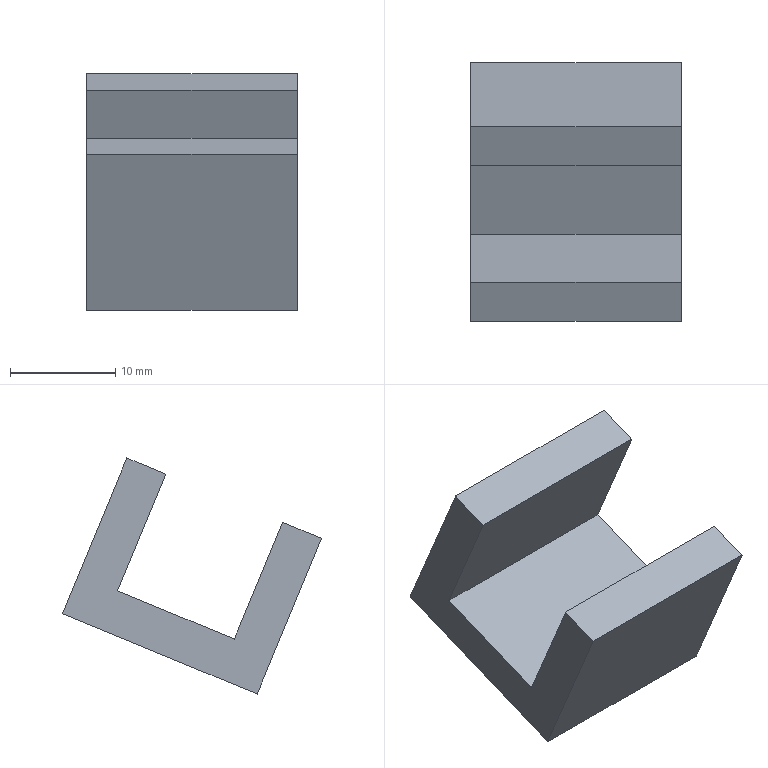Component | SolidWorks | 2026.08.03FixedRail-1 | 1 solid | 10 faces | box 20 x 24.59 x 22.42 mm | volume 3520 mm3 | plane 10
build123d program:
from build123d import *

# Parameters (mm, degrees)
BOSS_EXTRUDE2_DEPTH = 10


with BuildPart() as part:
    # Sketch1 → Boss-Extrude2 (new, symmetric)
    with BuildSketch(Plane(origin=(0, 0, 0), x_dir=(0, 0, -1), z_dir=(1, 0, 0))):
        Polygon((-16, 10), (0, 10), (0, -10), (-16, -10), (-16, -6), (-4, -6), (-4, 6), (-16, 6), align=None)
    extrude(amount=BOSS_EXTRUDE2_DEPTH, both=True)


solid = part.part

# Placed as in the assembly
solid = solid.moved(Location((80.094, 7.464, 7.823), (22.448, 0, 0)))
STEP:
#1=COLOUR_RGB('',0.7922,0.8196,0.9333);
#2=FILL_AREA_STYLE_COLOUR('',#1);
#3=FILL_AREA_STYLE('',(#2));
#4=SURFACE_STYLE_FILL_AREA(#3);
#5=SURFACE_SIDE_STYLE('',(#4));
#6=SURFACE_STYLE_USAGE(.BOTH.,#5);
#7=PRESENTATION_STYLE_ASSIGNMENT((#6));
#8=CARTESIAN_POINT('',(2.76,0.4172,1.041));
#9=VERTEX_POINT('',#8);
#10=CARTESIAN_POINT('',(2.76,0.2716,0.9804));
#11=VERTEX_POINT('',#10);
#12=CARTESIAN_POINT('',(2.76,0.4172,1.041));
#13=DIRECTION('',(0.,-0.9242,-0.3818));
#14=VECTOR('',#13,39.37);
#15=LINE('',#12,#14);
#16=EDGE_CURVE('',#9,#11,#15,.T.);
#17=ORIENTED_EDGE('',*,*,#16,.T.);
#18=CARTESIAN_POINT('',(3.547,0.2716,0.9804));
#19=VERTEX_POINT('',#18);
#20=CARTESIAN_POINT('',(3.547,0.2716,0.9804));
#21=DIRECTION('',(-1.,0.,0.));
#22=VECTOR('',#21,39.37);
#23=LINE('',#20,#22);
#24=EDGE_CURVE('',#19,#11,#23,.T.);
#25=ORIENTED_EDGE('',*,*,#24,.F.);
#26=CARTESIAN_POINT('',(3.547,0.4172,1.041));
#27=VERTEX_POINT('',#26);
#28=CARTESIAN_POINT('',(3.547,0.4172,1.041));
#29=DIRECTION('',(0.,-0.9242,-0.3818));
#30=VECTOR('',#29,39.37);
#31=LINE('',#28,#30);
#32=EDGE_CURVE('',#27,#19,#31,.T.);
#33=ORIENTED_EDGE('',*,*,#32,.F.);
#34=CARTESIAN_POINT('',(3.547,0.4172,1.041));
#35=DIRECTION('',(-1.,0.,0.));
#36=VECTOR('',#35,39.37);
#37=LINE('',#34,#36);
#38=EDGE_CURVE('',#27,#9,#37,.T.);
#39=ORIENTED_EDGE('',*,*,#38,.T.);
#40=EDGE_LOOP('',(#17,#25,#33,#39));
#41=FACE_OUTER_BOUND('',#40,.T.);
#42=CARTESIAN_POINT('',(3.547,0.4172,1.041));
#43=DIRECTION('',(0.,0.3818,-0.9242));
#44=DIRECTION('',(-1.,0.,0.));
#45=AXIS2_PLACEMENT_3D('',#42,#43,#44);
#46=PLANE('',#45);
#47=ADVANCED_FACE('',(#41),#46,.F.);
#48=CARTESIAN_POINT('',(2.76,0.452,0.5437));
#49=VERTEX_POINT('',#48);
#50=CARTESIAN_POINT('',(2.76,0.2716,0.9804));
#51=DIRECTION('',(0.,0.3818,-0.9242));
#52=VECTOR('',#51,39.37);
#53=LINE('',#50,#52);
#54=EDGE_CURVE('',#11,#49,#53,.T.);
#55=ORIENTED_EDGE('',*,*,#54,.T.);
#56=CARTESIAN_POINT('',(3.547,0.452,0.5437));
#57=VERTEX_POINT('',#56);
#58=CARTESIAN_POINT('',(3.547,0.452,0.5437));
#59=DIRECTION('',(-1.,0.,0.));
#60=VECTOR('',#59,39.37);
#61=LINE('',#58,#60);
#62=EDGE_CURVE('',#57,#49,#61,.T.);
#63=ORIENTED_EDGE('',*,*,#62,.F.);
#64=CARTESIAN_POINT('',(3.547,0.2716,0.9804));
#65=DIRECTION('',(0.,0.3818,-0.9242));
#66=VECTOR('',#65,39.37);
#67=LINE('',#64,#66);
#68=EDGE_CURVE('',#19,#57,#67,.T.);
#69=ORIENTED_EDGE('',*,*,#68,.F.);
#70=ORIENTED_EDGE('',*,*,#24,.T.);
#71=EDGE_LOOP('',(#55,#63,#69,#70));
#72=FACE_OUTER_BOUND('',#71,.T.);
#73=CARTESIAN_POINT('',(3.547,0.2716,0.9804));
#74=DIRECTION('',(0.,0.9242,0.3818));
#75=DIRECTION('',(0.,-0.3818,0.9242));
#76=AXIS2_PLACEMENT_3D('',#73,#74,#75);
#77=PLANE('',#76);
#78=ADVANCED_FACE('',(#72),#77,.F.);
#79=CARTESIAN_POINT('',(2.76,0.01541,0.3633));
#80=VERTEX_POINT('',#79);
#81=CARTESIAN_POINT('',(2.76,0.452,0.5437));
#82=DIRECTION('',(0.,-0.9242,-0.3818));
#83=VECTOR('',#82,39.37);
#84=LINE('',#81,#83);
#85=EDGE_CURVE('',#49,#80,#84,.T.);
#86=ORIENTED_EDGE('',*,*,#85,.T.);
#87=CARTESIAN_POINT('',(3.547,0.01541,0.3633));
#88=VERTEX_POINT('',#87);
#89=CARTESIAN_POINT('',(3.547,0.01541,0.3633));
#90=DIRECTION('',(-1.,0.,0.));
#91=VECTOR('',#90,39.37);
#92=LINE('',#89,#91);
#93=EDGE_CURVE('',#88,#80,#92,.T.);
#94=ORIENTED_EDGE('',*,*,#93,.F.);
#95=CARTESIAN_POINT('',(3.547,0.452,0.5437));
#96=DIRECTION('',(0.,-0.9242,-0.3818));
#97=VECTOR('',#96,39.37);
#98=LINE('',#95,#97);
#99=EDGE_CURVE('',#57,#88,#98,.T.);
#100=ORIENTED_EDGE('',*,*,#99,.F.);
#101=ORIENTED_EDGE('',*,*,#62,.T.);
#102=EDGE_LOOP('',(#86,#94,#100,#101));
#103=FACE_OUTER_BOUND('',#102,.T.);
#104=CARTESIAN_POINT('',(3.547,0.452,0.5437));
#105=DIRECTION('',(0.,0.3818,-0.9242));
#106=DIRECTION('',(0.,0.9242,0.3818));
#107=AXIS2_PLACEMENT_3D('',#104,#105,#106);
#108=PLANE('',#107);
#109=ADVANCED_FACE('',(#103),#108,.F.);
#110=CARTESIAN_POINT('',(2.76,-0.165,0.8));
#111=VERTEX_POINT('',#110);
#112=CARTESIAN_POINT('',(2.76,0.01541,0.3633));
#113=DIRECTION('',(0.,-0.3818,0.9242));
#114=VECTOR('',#113,39.37);
#115=LINE('',#112,#114);
#116=EDGE_CURVE('',#80,#111,#115,.T.);
#117=ORIENTED_EDGE('',*,*,#116,.T.);
#118=CARTESIAN_POINT('',(3.547,-0.165,0.8));
#119=VERTEX_POINT('',#118);
#120=CARTESIAN_POINT('',(3.547,-0.165,0.8));
#121=DIRECTION('',(-1.,0.,0.));
#122=VECTOR('',#121,39.37);
#123=LINE('',#120,#122);
#124=EDGE_CURVE('',#119,#111,#123,.T.);
#125=ORIENTED_EDGE('',*,*,#124,.F.);
#126=CARTESIAN_POINT('',(3.547,0.01541,0.3633));
#127=DIRECTION('',(0.,-0.3818,0.9242));
#128=VECTOR('',#127,39.37);
#129=LINE('',#126,#128);
#130=EDGE_CURVE('',#88,#119,#129,.T.);
#131=ORIENTED_EDGE('',*,*,#130,.F.);
#132=ORIENTED_EDGE('',*,*,#93,.T.);
#133=EDGE_LOOP('',(#117,#125,#131,#132));
#134=FACE_OUTER_BOUND('',#133,.T.);
#135=CARTESIAN_POINT('',(3.547,0.01541,0.3633));
#136=DIRECTION('',(0.,-0.9242,-0.3818));
#137=DIRECTION('',(0.,0.3818,-0.9242));
#138=AXIS2_PLACEMENT_3D('',#135,#136,#137);
#139=PLANE('',#138);
#140=ADVANCED_FACE('',(#134),#139,.F.);
#141=CARTESIAN_POINT('',(2.76,-0.3105,0.7399));
#142=VERTEX_POINT('',#141);
#143=CARTESIAN_POINT('',(2.76,-0.165,0.8));
#144=DIRECTION('',(0.,-0.9242,-0.3818));
#145=VECTOR('',#144,39.37);
#146=LINE('',#143,#145);
#147=EDGE_CURVE('',#111,#142,#146,.T.);
#148=ORIENTED_EDGE('',*,*,#147,.T.);
#149=CARTESIAN_POINT('',(3.547,-0.3105,0.7399));
#150=VERTEX_POINT('',#149);
#151=CARTESIAN_POINT('',(3.547,-0.3105,0.7399));
#152=DIRECTION('',(-1.,0.,0.));
#153=VECTOR('',#152,39.37);
#154=LINE('',#151,#153);
#155=EDGE_CURVE('',#150,#142,#154,.T.);
#156=ORIENTED_EDGE('',*,*,#155,.F.);
#157=CARTESIAN_POINT('',(3.547,-0.165,0.8));
#158=DIRECTION('',(0.,-0.9242,-0.3818));
#159=VECTOR('',#158,39.37);
#160=LINE('',#157,#159);
#161=EDGE_CURVE('',#119,#150,#160,.T.);
#162=ORIENTED_EDGE('',*,*,#161,.F.);
#163=ORIENTED_EDGE('',*,*,#124,.T.);
#164=EDGE_LOOP('',(#148,#156,#162,#163));
#165=FACE_OUTER_BOUND('',#164,.T.);
#166=CARTESIAN_POINT('',(3.547,-0.165,0.8));
#167=DIRECTION('',(0.,0.3818,-0.9242));
#168=DIRECTION('',(-1.,0.,0.));
#169=AXIS2_PLACEMENT_3D('',#166,#167,#168);
#170=PLANE('',#169);
#171=ADVANCED_FACE('',(#165),#170,.F.);
#172=CARTESIAN_POINT('',(2.76,-0.07001,0.1577));
#173=VERTEX_POINT('',#172);
#174=CARTESIAN_POINT('',(2.76,-0.07001,0.1577));
#175=DIRECTION('',(0.,0.3818,-0.9242));
#176=VECTOR('',#175,39.37);
#177=LINE('',#174,#176);
#178=EDGE_CURVE('',#142,#173,#177,.T.);
#179=ORIENTED_EDGE('',*,*,#178,.T.);
#180=CARTESIAN_POINT('',(3.547,-0.07001,0.1577));
#181=VERTEX_POINT('',#180);
#182=CARTESIAN_POINT('',(3.547,-0.07001,0.1577));
#183=DIRECTION('',(-1.,0.,0.));
#184=VECTOR('',#183,39.37);
#185=LINE('',#182,#184);
#186=EDGE_CURVE('',#181,#173,#185,.T.);
#187=ORIENTED_EDGE('',*,*,#186,.F.);
#188=CARTESIAN_POINT('',(3.547,-0.07001,0.1577));
#189=DIRECTION('',(0.,0.3818,-0.9242));
#190=VECTOR('',#189,39.37);
#191=LINE('',#188,#190);
#192=EDGE_CURVE('',#150,#181,#191,.T.);
#193=ORIENTED_EDGE('',*,*,#192,.F.);
#194=ORIENTED_EDGE('',*,*,#155,.T.);
#195=EDGE_LOOP('',(#179,#187,#193,#194));
#196=FACE_OUTER_BOUND('',#195,.T.);
#197=CARTESIAN_POINT('',(3.547,-0.07001,0.1577));
#198=DIRECTION('',(0.,0.9242,0.3818));
#199=DIRECTION('',(0.,-0.3818,0.9242));
#200=AXIS2_PLACEMENT_3D('',#197,#198,#199);
#201=PLANE('',#200);
#202=ADVANCED_FACE('',(#196),#201,.F.);
#203=CARTESIAN_POINT('',(2.76,0.6577,0.4583));
#204=VERTEX_POINT('',#203);
#205=CARTESIAN_POINT('',(2.76,0.6577,0.4583));
#206=DIRECTION('',(0.,0.9242,0.3818));
#207=VECTOR('',#206,39.37);
#208=LINE('',#205,#207);
#209=EDGE_CURVE('',#173,#204,#208,.T.);
#210=ORIENTED_EDGE('',*,*,#209,.T.);
#211=CARTESIAN_POINT('',(3.547,0.6577,0.4583));
#212=VERTEX_POINT('',#211);
#213=CARTESIAN_POINT('',(3.547,0.6577,0.4583));
#214=DIRECTION('',(-1.,0.,0.));
#215=VECTOR('',#214,39.37);
#216=LINE('',#213,#215);
#217=EDGE_CURVE('',#212,#204,#216,.T.);
#218=ORIENTED_EDGE('',*,*,#217,.F.);
#219=CARTESIAN_POINT('',(3.547,0.6577,0.4583));
#220=DIRECTION('',(0.,0.9242,0.3818));
#221=VECTOR('',#220,39.37);
#222=LINE('',#219,#221);
#223=EDGE_CURVE('',#181,#212,#222,.T.);
#224=ORIENTED_EDGE('',*,*,#223,.F.);
#225=ORIENTED_EDGE('',*,*,#186,.T.);
#226=EDGE_LOOP('',(#210,#218,#224,#225));
#227=FACE_OUTER_BOUND('',#226,.T.);
#228=CARTESIAN_POINT('',(3.547,0.6577,0.4583));
#229=DIRECTION('',(0.,-0.3818,0.9242));
#230=DIRECTION('',(1.,0.,0.));
#231=AXIS2_PLACEMENT_3D('',#228,#229,#230);
#232=PLANE('',#231);
#233=ADVANCED_FACE('',(#227),#232,.F.);
#234=CARTESIAN_POINT('',(2.76,0.4172,1.041));
#235=DIRECTION('',(0.,-0.3818,0.9242));
#236=VECTOR('',#235,39.37);
#237=LINE('',#234,#236);
#238=EDGE_CURVE('',#204,#9,#237,.T.);
#239=ORIENTED_EDGE('',*,*,#238,.T.);
#240=ORIENTED_EDGE('',*,*,#38,.F.);
#241=CARTESIAN_POINT('',(3.547,0.4172,1.041));
#242=DIRECTION('',(0.,-0.3818,0.9242));
#243=VECTOR('',#242,39.37);
#244=LINE('',#241,#243);
#245=EDGE_CURVE('',#212,#27,#244,.T.);
#246=ORIENTED_EDGE('',*,*,#245,.F.);
#247=ORIENTED_EDGE('',*,*,#217,.T.);
#248=EDGE_LOOP('',(#239,#240,#246,#247));
#249=FACE_OUTER_BOUND('',#248,.T.);
#250=CARTESIAN_POINT('',(3.547,0.4172,1.041));
#251=DIRECTION('',(0.,-0.9242,-0.3818));
#252=DIRECTION('',(0.,0.3818,-0.9242));
#253=AXIS2_PLACEMENT_3D('',#250,#251,#252);
#254=PLANE('',#253);
#255=ADVANCED_FACE('',(#249),#254,.F.);
#256=ORIENTED_EDGE('',*,*,#32,.T.);
#257=ORIENTED_EDGE('',*,*,#68,.T.);
#258=ORIENTED_EDGE('',*,*,#99,.T.);
#259=ORIENTED_EDGE('',*,*,#130,.T.);
#260=ORIENTED_EDGE('',*,*,#161,.T.);
#261=ORIENTED_EDGE('',*,*,#192,.T.);
#262=ORIENTED_EDGE('',*,*,#223,.T.);
#263=ORIENTED_EDGE('',*,*,#245,.T.);
#264=EDGE_LOOP('',(#256,#257,#258,#259,#260,#261,#262,#263));
#265=FACE_OUTER_BOUND('',#264,.T.);
#266=CARTESIAN_POINT('',(3.547,0.2939,0.308));
#267=DIRECTION('',(1.,0.,0.));
#268=DIRECTION('',(0.,0.3818,-0.9242));
#269=AXIS2_PLACEMENT_3D('',#266,#267,#268);
#270=PLANE('',#269);
#271=ADVANCED_FACE('',(#265),#270,.T.);
#272=ORIENTED_EDGE('',*,*,#16,.F.);
#273=ORIENTED_EDGE('',*,*,#238,.F.);
#274=ORIENTED_EDGE('',*,*,#209,.F.);
#275=ORIENTED_EDGE('',*,*,#178,.F.);
#276=ORIENTED_EDGE('',*,*,#147,.F.);
#277=ORIENTED_EDGE('',*,*,#116,.F.);
#278=ORIENTED_EDGE('',*,*,#85,.F.);
#279=ORIENTED_EDGE('',*,*,#54,.F.);
#280=EDGE_LOOP('',(#272,#273,#274,#275,#276,#277,#278,#279));
#281=FACE_OUTER_BOUND('',#280,.T.);
#282=CARTESIAN_POINT('',(2.76,0.2939,0.308));
#283=DIRECTION('',(1.,0.,0.));
#284=DIRECTION('',(0.,0.3818,-0.9242));
#285=AXIS2_PLACEMENT_3D('',#282,#283,#284);
#286=PLANE('',#285);
#287=ADVANCED_FACE('',(#281),#286,.F.);
#288=CLOSED_SHELL('',(#47,#78,#109,#140,#171,#202,#233,#255,#271,#287));
#289=MANIFOLD_SOLID_BREP('',#288);
#290=STYLED_ITEM('',(#7),#289);
#291=(LENGTH_UNIT()NAMED_UNIT(*)SI_UNIT($,.METRE.));
#292=LENGTH_MEASURE_WITH_UNIT(LENGTH_MEASURE(0.0254),#291);
#293=DIMENSIONAL_EXPONENTS(1.,0.,0.,0.,0.,0.,0.);
#294=(CONVERSION_BASED_UNIT('',#292)LENGTH_UNIT()NAMED_UNIT(#293));
#295=UNCERTAINTY_MEASURE_WITH_UNIT(LENGTH_MEASURE(0.00001),#294,'','');
#296=(NAMED_UNIT(*)PLANE_ANGLE_UNIT()SI_UNIT($,.RADIAN.));
#297=(NAMED_UNIT(*)SI_UNIT($,.STERADIAN.)SOLID_ANGLE_UNIT());
#298=(GEOMETRIC_REPRESENTATION_CONTEXT(3)GLOBAL_UNCERTAINTY_ASSIGNED_CONTEXT((#295))GLOBAL_UNIT_ASSIGNED_CONTEXT((#294,#296,#297))REPRESENTATION_CONTEXT('',''));
#299=MECHANICAL_DESIGN_GEOMETRIC_PRESENTATION_REPRESENTATION('',(#290),#298);
#300=PRESENTATION_LAYER_ASSIGNMENT('','',(#290));
#301=CARTESIAN_POINT('',(0.,0.,0.));
#302=DIRECTION('',(0.,0.,1.));
#303=DIRECTION('',(1.,0.,0.));
#304=AXIS2_PLACEMENT_3D('',#301,#302,#303);
#305=(LENGTH_UNIT()NAMED_UNIT(*)SI_UNIT($,.METRE.));
#306=LENGTH_MEASURE_WITH_UNIT(LENGTH_MEASURE(0.0254),#305);
#307=DIMENSIONAL_EXPONENTS(1.,0.,0.,0.,0.,0.,0.);
#308=(CONVERSION_BASED_UNIT('',#306)LENGTH_UNIT()NAMED_UNIT(#307));
#309=UNCERTAINTY_MEASURE_WITH_UNIT(LENGTH_MEASURE(0.00001),#308,'','');
#310=(NAMED_UNIT(*)PLANE_ANGLE_UNIT()SI_UNIT($,.RADIAN.));
#311=(NAMED_UNIT(*)SI_UNIT($,.STERADIAN.)SOLID_ANGLE_UNIT());
#312=(GEOMETRIC_REPRESENTATION_CONTEXT(3)GLOBAL_UNCERTAINTY_ASSIGNED_CONTEXT((#309))GLOBAL_UNIT_ASSIGNED_CONTEXT((#308,#310,#311))REPRESENTATION_CONTEXT('',''));
#313=ADVANCED_BREP_SHAPE_REPRESENTATION('',(#289,#304),#312);